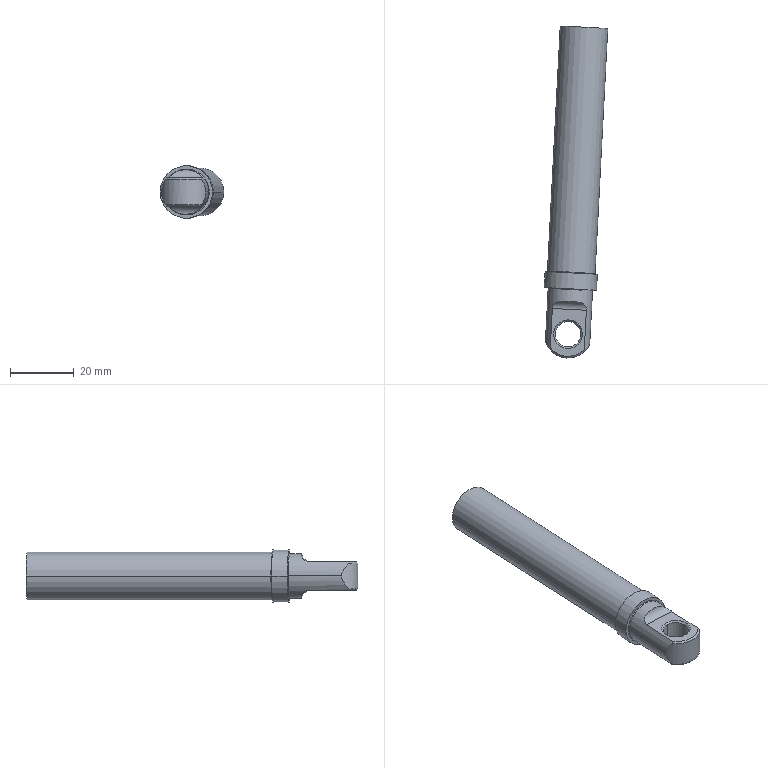Component | SolidWorks | CylinderBarrel-1 | 1 solid | 28 faces | box 20.01 x 104.57 x 16.5 mm | volume 13001 mm3 | cylinder 13 | plane 6 | cone 5 | torus 4 | commonest cylinder face diameters 8 x4 15 x3 14 x2 16.5 x2 5 x2
STEP:
#1=COLOUR_RGB('',0.7922,0.8196,0.9333);
#2=FILL_AREA_STYLE_COLOUR('',#1);
#3=FILL_AREA_STYLE('',(#2));
#4=SURFACE_STYLE_FILL_AREA(#3);
#5=SURFACE_SIDE_STYLE('',(#4));
#6=SURFACE_STYLE_USAGE(.BOTH.,#5);
#7=PRESENTATION_STYLE_ASSIGNMENT((#6));
#8=CARTESIAN_POINT('',(4.187,-5.913,6.691));
#9=VERTEX_POINT('',#8);
#10=CARTESIAN_POINT('',(4.738,-5.942,6.691));
#11=VERTEX_POINT('',#10);
#12=CARTESIAN_POINT('',(4.462,-5.928,6.691));
#13=DIRECTION('',(-0.0519,-0.9987,0.));
#14=DIRECTION('',(0.9987,-0.0519,0.));
#15=AXIS2_PLACEMENT_3D('',#12,#13,#14);
#16=CIRCLE('',#15,0.2756);
#17=EDGE_CURVE('',#9,#11,#16,.T.);
#18=ORIENTED_EDGE('',*,*,#17,.F.);
#19=CARTESIAN_POINT('',(4.178,-5.903,6.691));
#20=VERTEX_POINT('',#19);
#21=CARTESIAN_POINT('',(4.177,-5.913,6.691));
#22=DIRECTION('',(0.,0.,1.));
#23=DIRECTION('',(0.,-1.,0.));
#24=AXIS2_PLACEMENT_3D('',#21,#22,#23);
#25=CIRCLE('',#24,0.009843);
#26=EDGE_CURVE('',#9,#20,#25,.T.);
#27=ORIENTED_EDGE('',*,*,#26,.T.);
#28=CARTESIAN_POINT('',(4.748,-5.933,6.691));
#29=VERTEX_POINT('',#28);
#30=CARTESIAN_POINT('',(4.463,-5.918,6.691));
#31=DIRECTION('',(0.0519,0.9987,-0.));
#32=DIRECTION('',(0.9987,-0.0519,0.));
#33=AXIS2_PLACEMENT_3D('',#30,#31,#32);
#34=CIRCLE('',#33,0.2854);
#35=EDGE_CURVE('',#29,#20,#34,.T.);
#36=ORIENTED_EDGE('',*,*,#35,.F.);
#37=CARTESIAN_POINT('',(4.748,-5.942,6.691));
#38=DIRECTION('',(0.,-0.,-1.));
#39=DIRECTION('',(0.,1.,0.));
#40=AXIS2_PLACEMENT_3D('',#37,#38,#39);
#41=CIRCLE('',#40,0.009843);
#42=EDGE_CURVE('',#11,#29,#41,.T.);
#43=ORIENTED_EDGE('',*,*,#42,.F.);
#44=EDGE_LOOP('',(#18,#27,#36,#43));
#45=FACE_OUTER_BOUND('',#44,.T.);
#46=CARTESIAN_POINT('',(4.462,-5.928,6.691));
#47=DIRECTION('',(-0.0519,-0.9987,0.));
#48=DIRECTION('',(0.9987,-0.0519,-0.));
#49=AXIS2_PLACEMENT_3D('',#46,#47,#48);
#50=TOROIDAL_SURFACE('',#49,0.2854,0.009843);
#51=ADVANCED_FACE('',(#45),#50,.F.);
#52=CARTESIAN_POINT('',(4.168,-5.705,6.691));
#53=VERTEX_POINT('',#52);
#54=CARTESIAN_POINT('',(4.778,-5.737,6.691));
#55=VERTEX_POINT('',#54);
#56=CARTESIAN_POINT('',(4.473,-5.721,6.691));
#57=DIRECTION('',(-0.0519,-0.9987,0.));
#58=DIRECTION('',(0.9987,-0.0519,0.));
#59=AXIS2_PLACEMENT_3D('',#56,#57,#58);
#60=CIRCLE('',#59,0.3051);
#61=EDGE_CURVE('',#53,#55,#60,.T.);
#62=ORIENTED_EDGE('',*,*,#61,.F.);
#63=CARTESIAN_POINT('',(4.179,-5.696,6.691));
#64=VERTEX_POINT('',#63);
#65=CARTESIAN_POINT('',(4.169,-5.696,6.691));
#66=DIRECTION('',(0.,0.,1.));
#67=DIRECTION('',(0.,-1.,0.));
#68=AXIS2_PLACEMENT_3D('',#65,#66,#67);
#69=CIRCLE('',#68,0.009843);
#70=EDGE_CURVE('',#53,#64,#69,.T.);
#71=ORIENTED_EDGE('',*,*,#70,.T.);
#72=CARTESIAN_POINT('',(4.769,-5.727,6.691));
#73=VERTEX_POINT('',#72);
#74=CARTESIAN_POINT('',(4.474,-5.711,6.691));
#75=DIRECTION('',(0.0519,0.9987,-0.));
#76=DIRECTION('',(0.9987,-0.0519,0.));
#77=AXIS2_PLACEMENT_3D('',#74,#75,#76);
#78=CIRCLE('',#77,0.2953);
#79=EDGE_CURVE('',#73,#64,#78,.T.);
#80=ORIENTED_EDGE('',*,*,#79,.F.);
#81=CARTESIAN_POINT('',(4.778,-5.727,6.691));
#82=DIRECTION('',(0.,-0.,-1.));
#83=DIRECTION('',(0.,1.,0.));
#84=AXIS2_PLACEMENT_3D('',#81,#82,#83);
#85=CIRCLE('',#84,0.009843);
#86=EDGE_CURVE('',#55,#73,#85,.T.);
#87=ORIENTED_EDGE('',*,*,#86,.F.);
#88=EDGE_LOOP('',(#62,#71,#80,#87));
#89=FACE_OUTER_BOUND('',#88,.T.);
#90=CARTESIAN_POINT('',(4.474,-5.711,6.691));
#91=DIRECTION('',(-0.0519,-0.9987,0.));
#92=DIRECTION('',(0.9987,-0.0519,0.));
#93=AXIS2_PLACEMENT_3D('',#90,#91,#92);
#94=TOROIDAL_SURFACE('',#93,0.3051,0.009843);
#95=ADVANCED_FACE('',(#89),#94,.F.);
#96=CARTESIAN_POINT('',(4.419,-6.756,6.514));
#97=VERTEX_POINT('',#96);
#98=CARTESIAN_POINT('',(4.214,-6.646,6.514));
#99=VERTEX_POINT('',#98);
#100=CARTESIAN_POINT('',(4.434,-6.48,6.514));
#101=DIRECTION('',(0.,-0.,-1.));
#102=DIRECTION('',(-0.0519,-0.9987,0.));
#103=AXIS2_PLACEMENT_3D('',#100,#101,#102);
#104=CIRCLE('',#103,0.2756);
#105=EDGE_CURVE('',#97,#99,#104,.T.);
#106=ORIENTED_EDGE('',*,*,#105,.F.);
#107=CARTESIAN_POINT('',(4.418,-6.775,6.534));
#108=VERTEX_POINT('',#107);
#109=CARTESIAN_POINT('',(4.419,-6.756,6.514));
#110=DIRECTION('',(-0.0367,-0.7062,0.7071));
#111=VECTOR('',#110,39.37);
#112=LINE('',#109,#111);
#113=EDGE_CURVE('',#97,#108,#112,.T.);
#114=ORIENTED_EDGE('',*,*,#113,.T.);
#115=CARTESIAN_POINT('',(4.198,-6.658,6.534));
#116=VERTEX_POINT('',#115);
#117=CARTESIAN_POINT('',(4.434,-6.48,6.534));
#118=DIRECTION('',(-0.,0.,1.));
#119=DIRECTION('',(-0.0519,-0.9987,0.));
#120=AXIS2_PLACEMENT_3D('',#117,#118,#119);
#121=CIRCLE('',#120,0.2953);
#122=EDGE_CURVE('',#116,#108,#121,.T.);
#123=ORIENTED_EDGE('',*,*,#122,.F.);
#124=CARTESIAN_POINT('',(4.214,-6.646,6.514));
#125=CARTESIAN_POINT('',(4.208,-6.65,6.521));
#126=CARTESIAN_POINT('',(4.203,-6.654,6.527));
#127=CARTESIAN_POINT('',(4.198,-6.658,6.534));
#128=B_SPLINE_CURVE_WITH_KNOTS('',3,(#124,#125,#126,#127),.UNSPECIFIED.,.F.,.F.,(4,4),(0.,0.0007071),.UNSPECIFIED.);
#129=EDGE_CURVE('',#99,#116,#128,.T.);
#130=ORIENTED_EDGE('',*,*,#129,.F.);
#131=EDGE_LOOP('',(#106,#114,#123,#130));
#132=FACE_OUTER_BOUND('',#131,.T.);
#133=CARTESIAN_POINT('',(4.434,-6.48,6.514));
#134=DIRECTION('',(-0.,0.,1.));
#135=DIRECTION('',(-0.0519,-0.9987,0.));
#136=AXIS2_PLACEMENT_3D('',#133,#134,#135);
#137=CONICAL_SURFACE('',#136,0.2756,0.7854);
#138=ADVANCED_FACE('',(#132),#137,.T.);
#139=CARTESIAN_POINT('',(4.442,-6.323,6.849));
#140=VERTEX_POINT('',#139);
#141=CARTESIAN_POINT('',(4.426,-6.638,6.849));
#142=VERTEX_POINT('',#141);
#143=CARTESIAN_POINT('',(4.434,-6.48,6.849));
#144=DIRECTION('',(-0.,0.,1.));
#145=DIRECTION('',(0.0519,0.9987,0.));
#146=AXIS2_PLACEMENT_3D('',#143,#144,#145);
#147=CIRCLE('',#146,0.1575);
#148=EDGE_CURVE('',#140,#142,#147,.T.);
#149=ORIENTED_EDGE('',*,*,#148,.F.);
#150=CARTESIAN_POINT('',(4.443,-6.303,6.869));
#151=VERTEX_POINT('',#150);
#152=CARTESIAN_POINT('',(4.443,-6.303,6.869));
#153=DIRECTION('',(0.0367,0.7062,0.7071));
#154=VECTOR('',#153,39.37);
#155=LINE('',#152,#154);
#156=EDGE_CURVE('',#140,#151,#155,.T.);
#157=ORIENTED_EDGE('',*,*,#156,.T.);
#158=CARTESIAN_POINT('',(4.425,-6.657,6.869));
#159=VERTEX_POINT('',#158);
#160=CARTESIAN_POINT('',(4.434,-6.48,6.869));
#161=DIRECTION('',(0.,-0.,-1.));
#162=DIRECTION('',(0.0519,0.9987,0.));
#163=AXIS2_PLACEMENT_3D('',#160,#161,#162);
#164=CIRCLE('',#163,0.1772);
#165=EDGE_CURVE('',#159,#151,#164,.T.);
#166=ORIENTED_EDGE('',*,*,#165,.F.);
#167=CARTESIAN_POINT('',(4.425,-6.657,6.869));
#168=DIRECTION('',(-0.0367,-0.7062,0.7071));
#169=VECTOR('',#168,39.37);
#170=LINE('',#167,#169);
#171=EDGE_CURVE('',#142,#159,#170,.T.);
#172=ORIENTED_EDGE('',*,*,#171,.F.);
#173=EDGE_LOOP('',(#149,#157,#166,#172));
#174=FACE_OUTER_BOUND('',#173,.T.);
#175=CARTESIAN_POINT('',(4.434,-6.48,6.869));
#176=DIRECTION('',(-0.,0.,1.));
#177=DIRECTION('',(-0.0519,-0.9987,0.));
#178=AXIS2_PLACEMENT_3D('',#175,#176,#177);
#179=CONICAL_SURFACE('',#178,0.1772,0.7854);
#180=ADVANCED_FACE('',(#174),#179,.F.);
#181=CARTESIAN_POINT('',(4.442,-6.323,6.514));
#182=VERTEX_POINT('',#181);
#183=CARTESIAN_POINT('',(4.426,-6.638,6.514));
#184=VERTEX_POINT('',#183);
#185=CARTESIAN_POINT('',(4.434,-6.48,6.514));
#186=DIRECTION('',(-0.,0.,1.));
#187=DIRECTION('',(-0.0519,-0.9987,0.));
#188=AXIS2_PLACEMENT_3D('',#185,#186,#187);
#189=CIRCLE('',#188,0.1575);
#190=EDGE_CURVE('',#182,#184,#189,.T.);
#191=ORIENTED_EDGE('',*,*,#190,.F.);
#192=CARTESIAN_POINT('',(4.442,-6.323,6.298));
#193=DIRECTION('',(-0.,0.,1.));
#194=VECTOR('',#193,39.37);
#195=LINE('',#192,#194);
#196=EDGE_CURVE('',#182,#140,#195,.T.);
#197=ORIENTED_EDGE('',*,*,#196,.T.);
#198=ORIENTED_EDGE('',*,*,#148,.T.);
#199=CARTESIAN_POINT('',(4.426,-6.638,6.298));
#200=DIRECTION('',(-0.,0.,1.));
#201=VECTOR('',#200,39.37);
#202=LINE('',#199,#201);
#203=EDGE_CURVE('',#184,#142,#202,.T.);
#204=ORIENTED_EDGE('',*,*,#203,.F.);
#205=EDGE_LOOP('',(#191,#197,#198,#204));
#206=FACE_OUTER_BOUND('',#205,.T.);
#207=CARTESIAN_POINT('',(4.434,-6.48,6.298));
#208=DIRECTION('',(-0.,0.,1.));
#209=DIRECTION('',(-0.0519,-0.9987,0.));
#210=AXIS2_PLACEMENT_3D('',#207,#208,#209);
#211=CYLINDRICAL_SURFACE('',#210,0.1575);
#212=ADVANCED_FACE('',(#206),#211,.F.);
#213=CARTESIAN_POINT('',(4.65,-6.682,6.849));
#214=VERTEX_POINT('',#213);
#215=CARTESIAN_POINT('',(4.703,-6.6,6.691));
#216=VERTEX_POINT('',#215);
#217=CARTESIAN_POINT('',(4.65,-6.682,6.849));
#218=CARTESIAN_POINT('',(4.658,-6.673,6.838));
#219=CARTESIAN_POINT('',(4.665,-6.665,6.827));
#220=CARTESIAN_POINT('',(4.677,-6.648,6.804));
#221=CARTESIAN_POINT('',(4.683,-6.639,6.792));
#222=CARTESIAN_POINT('',(4.692,-6.623,6.766));
#223=CARTESIAN_POINT('',(4.696,-6.616,6.752));
#224=CARTESIAN_POINT('',(4.7,-6.607,6.73));
#225=CARTESIAN_POINT('',(4.702,-6.605,6.723));
#226=CARTESIAN_POINT('',(4.703,-6.601,6.707));
#227=CARTESIAN_POINT('',(4.703,-6.6,6.699));
#228=CARTESIAN_POINT('',(4.703,-6.6,6.691));
#229=B_SPLINE_CURVE_WITH_KNOTS('',3,(#217,#218,#219,#220,#221,#222,#223,#224,#225,#226,#227,#228),.UNSPECIFIED.,.F.,.F.,(4,2,2,2,2,4),(0.0007506,0.001947,0.003143,0.004339,0.004937,0.005535),.UNSPECIFIED.);
#230=EDGE_CURVE('',#214,#216,#229,.T.);
#231=ORIENTED_EDGE('',*,*,#230,.T.);
#232=CARTESIAN_POINT('',(4.73,-6.089,6.691));
#233=DIRECTION('',(0.0519,0.9987,-0.));
#234=VECTOR('',#233,39.37);
#235=LINE('',#232,#234);
#236=EDGE_CURVE('',#216,#11,#235,.T.);
#237=ORIENTED_EDGE('',*,*,#236,.T.);
#238=CARTESIAN_POINT('',(4.462,-5.928,6.691));
#239=DIRECTION('',(-0.0519,-0.9987,0.));
#240=DIRECTION('',(0.9987,-0.0519,0.));
#241=AXIS2_PLACEMENT_3D('',#238,#239,#240);
#242=CIRCLE('',#241,0.2756);
#243=EDGE_CURVE('',#11,#9,#242,.T.);
#244=ORIENTED_EDGE('',*,*,#243,.T.);
#245=CARTESIAN_POINT('',(4.153,-6.572,6.691));
#246=VERTEX_POINT('',#245);
#247=CARTESIAN_POINT('',(4.18,-6.061,6.691));
#248=DIRECTION('',(0.0519,0.9987,-0.));
#249=VECTOR('',#248,39.37);
#250=LINE('',#247,#249);
#251=EDGE_CURVE('',#246,#9,#250,.T.);
#252=ORIENTED_EDGE('',*,*,#251,.F.);
#253=CARTESIAN_POINT('',(4.198,-6.658,6.849));
#254=VERTEX_POINT('',#253);
#255=CARTESIAN_POINT('',(4.153,-6.572,6.691));
#256=CARTESIAN_POINT('',(4.153,-6.572,6.699));
#257=CARTESIAN_POINT('',(4.153,-6.573,6.707));
#258=CARTESIAN_POINT('',(4.154,-6.576,6.723));
#259=CARTESIAN_POINT('',(4.155,-6.579,6.73));
#260=CARTESIAN_POINT('',(4.159,-6.588,6.752));
#261=CARTESIAN_POINT('',(4.162,-6.595,6.766));
#262=CARTESIAN_POINT('',(4.169,-6.612,6.792));
#263=CARTESIAN_POINT('',(4.174,-6.621,6.804));
#264=CARTESIAN_POINT('',(4.185,-6.64,6.827));
#265=CARTESIAN_POINT('',(4.191,-6.649,6.838));
#266=CARTESIAN_POINT('',(4.198,-6.658,6.849));
#267=B_SPLINE_CURVE_WITH_KNOTS('',3,(#255,#256,#257,#258,#259,#260,#261,#262,#263,#264,#265,#266),.UNSPECIFIED.,.F.,.F.,(4,2,2,2,2,4),(0.005535,0.006132,0.006728,0.007922,0.009116,0.01031),.UNSPECIFIED.);
#268=EDGE_CURVE('',#246,#254,#267,.T.);
#269=ORIENTED_EDGE('',*,*,#268,.T.);
#270=CARTESIAN_POINT('',(4.214,-6.646,6.869));
#271=VERTEX_POINT('',#270);
#272=CARTESIAN_POINT('',(4.198,-6.658,6.849));
#273=CARTESIAN_POINT('',(4.203,-6.654,6.855));
#274=CARTESIAN_POINT('',(4.208,-6.65,6.862));
#275=CARTESIAN_POINT('',(4.214,-6.646,6.869));
#276=B_SPLINE_CURVE_WITH_KNOTS('',3,(#272,#273,#274,#275),.UNSPECIFIED.,.F.,.F.,(4,4),(0.,0.0007071),.UNSPECIFIED.);
#277=EDGE_CURVE('',#254,#271,#276,.T.);
#278=ORIENTED_EDGE('',*,*,#277,.T.);
#279=CARTESIAN_POINT('',(4.239,-6.162,6.869));
#280=VERTEX_POINT('',#279);
#281=CARTESIAN_POINT('',(4.217,-6.575,6.869));
#282=DIRECTION('',(0.0519,0.9987,-0.));
#283=VECTOR('',#282,39.37);
#284=LINE('',#281,#283);
#285=EDGE_CURVE('',#271,#280,#284,.T.);
#286=ORIENTED_EDGE('',*,*,#285,.T.);
#287=CARTESIAN_POINT('',(4.661,-6.184,6.869));
#288=VERTEX_POINT('',#287);
#289=CARTESIAN_POINT('',(4.239,-6.162,6.869));
#290=CARTESIAN_POINT('',(4.239,-6.156,6.869));
#291=CARTESIAN_POINT('',(4.24,-6.15,6.869));
#292=CARTESIAN_POINT('',(4.242,-6.139,6.871));
#293=CARTESIAN_POINT('',(4.244,-6.133,6.873));
#294=CARTESIAN_POINT('',(4.25,-6.117,6.879));
#295=CARTESIAN_POINT('',(4.256,-6.108,6.885));
#296=CARTESIAN_POINT('',(4.267,-6.097,6.895));
#297=CARTESIAN_POINT('',(4.271,-6.094,6.898));
#298=CARTESIAN_POINT('',(4.279,-6.088,6.905));
#299=CARTESIAN_POINT('',(4.284,-6.086,6.908));
#300=CARTESIAN_POINT('',(4.293,-6.082,6.915));
#301=CARTESIAN_POINT('',(4.297,-6.08,6.918));
#302=CARTESIAN_POINT('',(4.307,-6.077,6.925));
#303=CARTESIAN_POINT('',(4.312,-6.076,6.928));
#304=CARTESIAN_POINT('',(4.328,-6.073,6.936));
#305=CARTESIAN_POINT('',(4.339,-6.072,6.942));
#306=CARTESIAN_POINT('',(4.361,-6.071,6.951));
#307=CARTESIAN_POINT('',(4.372,-6.071,6.955));
#308=CARTESIAN_POINT('',(4.395,-6.072,6.961));
#309=CARTESIAN_POINT('',(4.407,-6.073,6.963));
#310=CARTESIAN_POINT('',(4.431,-6.074,6.966));
#311=CARTESIAN_POINT('',(4.443,-6.074,6.967));
#312=CARTESIAN_POINT('',(4.479,-6.076,6.967));
#313=CARTESIAN_POINT('',(4.503,-6.077,6.964));
#314=CARTESIAN_POINT('',(4.537,-6.08,6.955));
#315=CARTESIAN_POINT('',(4.549,-6.081,6.951));
#316=CARTESIAN_POINT('',(4.571,-6.084,6.942));
#317=CARTESIAN_POINT('',(4.581,-6.086,6.936));
#318=CARTESIAN_POINT('',(4.602,-6.092,6.925));
#319=CARTESIAN_POINT('',(4.611,-6.096,6.918));
#320=CARTESIAN_POINT('',(4.628,-6.106,6.905));
#321=CARTESIAN_POINT('',(4.636,-6.112,6.898));
#322=CARTESIAN_POINT('',(4.646,-6.124,6.888));
#323=CARTESIAN_POINT('',(4.648,-6.129,6.885));
#324=CARTESIAN_POINT('',(4.653,-6.139,6.879));
#325=CARTESIAN_POINT('',(4.655,-6.144,6.877));
#326=CARTESIAN_POINT('',(4.658,-6.155,6.873));
#327=CARTESIAN_POINT('',(4.659,-6.16,6.871));
#328=CARTESIAN_POINT('',(4.661,-6.172,6.869));
#329=CARTESIAN_POINT('',(4.661,-6.178,6.869));
#330=CARTESIAN_POINT('',(4.661,-6.184,6.869));
#331=B_SPLINE_CURVE_WITH_KNOTS('',3,(#289,#290,#291,#292,#293,#294,#295,#296,#297,#298,#299,#300,#301,#302,#303,#304,#305,#306,#307,#308,#309,#310,#311,#312,#313,#314,#315,#316,#317,#318,#319,#320,#321,#322,#323,#324,#325,#326,#327,#328,#329,#330),.UNSPECIFIED.,.F.,.F.,(4,2,2,2,2,2,2,2,2,2,2,2,2,2,2,2,2,2,2,2,4),(0.,0.0004585,0.000917,0.001834,0.002292,0.002751,0.003209,0.003668,0.004585,0.005502,0.006419,0.007336,0.00917,0.01009,0.011,0.01192,0.01284,0.0133,0.01375,0.01421,0.01467),.UNSPECIFIED.);
#332=EDGE_CURVE('',#280,#288,#331,.T.);
#333=ORIENTED_EDGE('',*,*,#332,.T.);
#334=CARTESIAN_POINT('',(4.635,-6.668,6.869));
#335=VERTEX_POINT('',#334);
#336=CARTESIAN_POINT('',(4.639,-6.597,6.869));
#337=DIRECTION('',(0.0519,0.9987,-0.));
#338=VECTOR('',#337,39.37);
#339=LINE('',#336,#338);
#340=EDGE_CURVE('',#335,#288,#339,.T.);
#341=ORIENTED_EDGE('',*,*,#340,.F.);
#342=CARTESIAN_POINT('',(4.635,-6.668,6.869));
#343=CARTESIAN_POINT('',(4.641,-6.672,6.862));
#344=CARTESIAN_POINT('',(4.645,-6.677,6.855));
#345=CARTESIAN_POINT('',(4.65,-6.682,6.849));
#346=B_SPLINE_CURVE_WITH_KNOTS('',3,(#342,#343,#344,#345),.UNSPECIFIED.,.F.,.F.,(4,4),(0.,0.0007071),.UNSPECIFIED.);
#347=EDGE_CURVE('',#335,#214,#346,.T.);
#348=ORIENTED_EDGE('',*,*,#347,.T.);
#349=EDGE_LOOP('',(#231,#237,#244,#252,#269,#278,#286,#333,#341,#348));
#350=FACE_OUTER_BOUND('',#349,.T.);
#351=CARTESIAN_POINT('',(4.455,-6.075,6.691));
#352=DIRECTION('',(0.0519,0.9987,-0.));
#353=DIRECTION('',(-0.9987,0.0519,0.));
#354=AXIS2_PLACEMENT_3D('',#351,#352,#353);
#355=CYLINDRICAL_SURFACE('',#354,0.2756);
#356=ADVANCED_FACE('',(#350),#355,.T.);
#357=CARTESIAN_POINT('',(4.787,-5.935,6.691));
#358=VERTEX_POINT('',#357);
#359=CARTESIAN_POINT('',(4.139,-5.901,6.691));
#360=VERTEX_POINT('',#359);
#361=CARTESIAN_POINT('',(4.463,-5.918,6.691));
#362=DIRECTION('',(-0.0519,-0.9987,0.));
#363=DIRECTION('',(0.9987,-0.0519,0.));
#364=AXIS2_PLACEMENT_3D('',#361,#362,#363);
#365=CIRCLE('',#364,0.3248);
#366=EDGE_CURVE('',#358,#360,#365,.T.);
#367=ORIENTED_EDGE('',*,*,#366,.F.);
#368=CARTESIAN_POINT('',(4.798,-5.738,6.691));
#369=VERTEX_POINT('',#368);
#370=CARTESIAN_POINT('',(4.787,-5.935,6.691));
#371=DIRECTION('',(0.0519,0.9987,-0.));
#372=VECTOR('',#371,39.37);
#373=LINE('',#370,#372);
#374=EDGE_CURVE('',#358,#369,#373,.T.);
#375=ORIENTED_EDGE('',*,*,#374,.T.);
#376=CARTESIAN_POINT('',(4.149,-5.704,6.691));
#377=VERTEX_POINT('',#376);
#378=CARTESIAN_POINT('',(4.473,-5.721,6.691));
#379=DIRECTION('',(-0.0519,-0.9987,0.));
#380=DIRECTION('',(0.9987,-0.0519,0.));
#381=AXIS2_PLACEMENT_3D('',#378,#379,#380);
#382=CIRCLE('',#381,0.3248);
#383=EDGE_CURVE('',#369,#377,#382,.T.);
#384=ORIENTED_EDGE('',*,*,#383,.T.);
#385=CARTESIAN_POINT('',(4.139,-5.901,6.691));
#386=DIRECTION('',(0.0519,0.9987,-0.));
#387=VECTOR('',#386,39.37);
#388=LINE('',#385,#387);
#389=EDGE_CURVE('',#360,#377,#388,.T.);
#390=ORIENTED_EDGE('',*,*,#389,.F.);
#391=EDGE_LOOP('',(#367,#375,#384,#390));
#392=FACE_OUTER_BOUND('',#391,.T.);
#393=CARTESIAN_POINT('',(4.463,-5.918,6.691));
#394=DIRECTION('',(0.0519,0.9987,-0.));
#395=DIRECTION('',(-0.9987,0.0519,0.));
#396=AXIS2_PLACEMENT_3D('',#393,#394,#395);
#397=CYLINDRICAL_SURFACE('',#396,0.3248);
#398=ADVANCED_FACE('',(#392),#397,.T.);
#399=CARTESIAN_POINT('',(4.316,-5.713,6.691));
#400=VERTEX_POINT('',#399);
#401=CARTESIAN_POINT('',(4.63,-5.729,6.691));
#402=VERTEX_POINT('',#401);
#403=CARTESIAN_POINT('',(4.473,-5.721,6.691));
#404=DIRECTION('',(-0.0519,-0.9987,0.));
#405=DIRECTION('',(0.9987,-0.0519,0.));
#406=AXIS2_PLACEMENT_3D('',#403,#404,#405);
#407=CIRCLE('',#406,0.1575);
#408=EDGE_CURVE('',#400,#402,#407,.T.);
#409=ORIENTED_EDGE('',*,*,#408,.T.);
#410=CARTESIAN_POINT('',(4.789,-2.682,6.691));
#411=VERTEX_POINT('',#410);
#412=CARTESIAN_POINT('',(4.63,-5.729,6.691));
#413=DIRECTION('',(0.0519,0.9987,-0.));
#414=VECTOR('',#413,39.37);
#415=LINE('',#412,#414);
#416=EDGE_CURVE('',#402,#411,#415,.T.);
#417=ORIENTED_EDGE('',*,*,#416,.T.);
#418=CARTESIAN_POINT('',(4.474,-2.666,6.691));
#419=VERTEX_POINT('',#418);
#420=CARTESIAN_POINT('',(4.632,-2.674,6.691));
#421=DIRECTION('',(-0.0519,-0.9987,0.));
#422=DIRECTION('',(0.9987,-0.0519,0.));
#423=AXIS2_PLACEMENT_3D('',#420,#421,#422);
#424=CIRCLE('',#423,0.1575);
#425=EDGE_CURVE('',#419,#411,#424,.T.);
#426=ORIENTED_EDGE('',*,*,#425,.F.);
#427=CARTESIAN_POINT('',(4.316,-5.713,6.691));
#428=DIRECTION('',(0.0519,0.9987,-0.));
#429=VECTOR('',#428,39.37);
#430=LINE('',#427,#429);
#431=EDGE_CURVE('',#400,#419,#430,.T.);
#432=ORIENTED_EDGE('',*,*,#431,.F.);
#433=EDGE_LOOP('',(#409,#417,#426,#432));
#434=FACE_OUTER_BOUND('',#433,.T.);
#435=CARTESIAN_POINT('',(4.473,-5.721,6.691));
#436=DIRECTION('',(0.0519,0.9987,-0.));
#437=DIRECTION('',(-0.9987,0.0519,0.));
#438=AXIS2_PLACEMENT_3D('',#435,#436,#437);
#439=CYLINDRICAL_SURFACE('',#438,0.1575);
#440=ADVANCED_FACE('',(#434),#439,.F.);
#441=CARTESIAN_POINT('',(4.474,-5.711,6.691));
#442=DIRECTION('',(0.0519,0.9987,-0.));
#443=DIRECTION('',(0.9987,-0.0519,0.));
#444=AXIS2_PLACEMENT_3D('',#441,#442,#443);
#445=CIRCLE('',#444,0.2953);
#446=EDGE_CURVE('',#64,#73,#445,.T.);
#447=ORIENTED_EDGE('',*,*,#446,.T.);
#448=CARTESIAN_POINT('',(4.926,-2.689,6.691));
#449=VERTEX_POINT('',#448);
#450=CARTESIAN_POINT('',(4.768,-5.737,6.691));
#451=DIRECTION('',(0.0519,0.9987,-0.));
#452=VECTOR('',#451,39.37);
#453=LINE('',#450,#452);
#454=EDGE_CURVE('',#73,#449,#453,.T.);
#455=ORIENTED_EDGE('',*,*,#454,.T.);
#456=CARTESIAN_POINT('',(4.337,-2.659,6.691));
#457=VERTEX_POINT('',#456);
#458=CARTESIAN_POINT('',(4.632,-2.674,6.691));
#459=DIRECTION('',(-0.0519,-0.9987,0.));
#460=DIRECTION('',(0.9987,-0.0519,0.));
#461=AXIS2_PLACEMENT_3D('',#458,#459,#460);
#462=CIRCLE('',#461,0.2953);
#463=EDGE_CURVE('',#449,#457,#462,.T.);
#464=ORIENTED_EDGE('',*,*,#463,.T.);
#465=CARTESIAN_POINT('',(4.178,-5.706,6.691));
#466=DIRECTION('',(0.0519,0.9987,-0.));
#467=VECTOR('',#466,39.37);
#468=LINE('',#465,#467);
#469=EDGE_CURVE('',#64,#457,#468,.T.);
#470=ORIENTED_EDGE('',*,*,#469,.F.);
#471=EDGE_LOOP('',(#447,#455,#464,#470));
#472=FACE_OUTER_BOUND('',#471,.T.);
#473=CARTESIAN_POINT('',(4.473,-5.721,6.691));
#474=DIRECTION('',(0.0519,0.9987,-0.));
#475=DIRECTION('',(-0.9987,0.0519,0.));
#476=AXIS2_PLACEMENT_3D('',#473,#474,#475);
#477=CYLINDRICAL_SURFACE('',#476,0.2953);
#478=ADVANCED_FACE('',(#472),#477,.T.);
#479=ORIENTED_EDGE('',*,*,#35,.T.);
#480=CARTESIAN_POINT('',(4.463,-5.918,6.691));
#481=DIRECTION('',(0.0519,0.9987,-0.));
#482=DIRECTION('',(0.9987,-0.0519,0.));
#483=AXIS2_PLACEMENT_3D('',#480,#481,#482);
#484=CIRCLE('',#483,0.2854);
#485=EDGE_CURVE('',#20,#29,#484,.T.);
#486=ORIENTED_EDGE('',*,*,#485,.T.);
#487=EDGE_LOOP('',(#479,#486));
#488=FACE_BOUND('',#487,.T.);
#489=CARTESIAN_POINT('',(4.463,-5.918,6.691));
#490=DIRECTION('',(-0.0519,-0.9987,0.));
#491=DIRECTION('',(0.9987,-0.0519,0.));
#492=AXIS2_PLACEMENT_3D('',#489,#490,#491);
#493=CIRCLE('',#492,0.3248);
#494=EDGE_CURVE('',#360,#358,#493,.T.);
#495=ORIENTED_EDGE('',*,*,#494,.T.);
#496=ORIENTED_EDGE('',*,*,#366,.T.);
#497=EDGE_LOOP('',(#495,#496));
#498=FACE_OUTER_BOUND('',#497,.T.);
#499=CARTESIAN_POINT('',(4.463,-5.918,6.691));
#500=DIRECTION('',(-0.0519,-0.9987,0.));
#501=DIRECTION('',(0.9987,-0.0519,0.));
#502=AXIS2_PLACEMENT_3D('',#499,#500,#501);
#503=PLANE('',#502);
#504=ADVANCED_FACE('',(#488,#498),#503,.T.);
#505=CARTESIAN_POINT('',(4.632,-2.674,6.691));
#506=DIRECTION('',(-0.0519,-0.9987,0.));
#507=DIRECTION('',(0.9987,-0.0519,0.));
#508=AXIS2_PLACEMENT_3D('',#505,#506,#507);
#509=CIRCLE('',#508,0.2953);
#510=EDGE_CURVE('',#457,#449,#509,.T.);
#511=ORIENTED_EDGE('',*,*,#510,.F.);
#512=ORIENTED_EDGE('',*,*,#463,.F.);
#513=EDGE_LOOP('',(#511,#512));
#514=FACE_OUTER_BOUND('',#513,.T.);
#515=ORIENTED_EDGE('',*,*,#425,.T.);
#516=CARTESIAN_POINT('',(4.632,-2.674,6.691));
#517=DIRECTION('',(-0.0519,-0.9987,0.));
#518=DIRECTION('',(0.9987,-0.0519,0.));
#519=AXIS2_PLACEMENT_3D('',#516,#517,#518);
#520=CIRCLE('',#519,0.1575);
#521=EDGE_CURVE('',#411,#419,#520,.T.);
#522=ORIENTED_EDGE('',*,*,#521,.T.);
#523=EDGE_LOOP('',(#515,#522));
#524=FACE_BOUND('',#523,.T.);
#525=CARTESIAN_POINT('',(4.632,-2.674,6.691));
#526=DIRECTION('',(-0.0519,-0.9987,0.));
#527=DIRECTION('',(0.9987,-0.0519,0.));
#528=AXIS2_PLACEMENT_3D('',#525,#526,#527);
#529=PLANE('',#528);
#530=ADVANCED_FACE('',(#514,#524),#529,.F.);
#531=ORIENTED_EDGE('',*,*,#454,.F.);
#532=ORIENTED_EDGE('',*,*,#79,.T.);
#533=ORIENTED_EDGE('',*,*,#469,.T.);
#534=ORIENTED_EDGE('',*,*,#510,.T.);
#535=EDGE_LOOP('',(#531,#532,#533,#534));
#536=FACE_OUTER_BOUND('',#535,.T.);
#537=CARTESIAN_POINT('',(4.473,-5.721,6.691));
#538=DIRECTION('',(0.0519,0.9987,-0.));
#539=DIRECTION('',(-0.9987,0.0519,0.));
#540=AXIS2_PLACEMENT_3D('',#537,#538,#539);
#541=CYLINDRICAL_SURFACE('',#540,0.2953);
#542=ADVANCED_FACE('',(#536),#541,.T.);
#543=ORIENTED_EDGE('',*,*,#416,.F.);
#544=CARTESIAN_POINT('',(4.473,-5.721,6.691));
#545=DIRECTION('',(-0.0519,-0.9987,0.));
#546=DIRECTION('',(0.9987,-0.0519,0.));
#547=AXIS2_PLACEMENT_3D('',#544,#545,#546);
#548=CIRCLE('',#547,0.1575);
#549=EDGE_CURVE('',#402,#400,#548,.T.);
#550=ORIENTED_EDGE('',*,*,#549,.T.);
#551=ORIENTED_EDGE('',*,*,#431,.T.);
#552=ORIENTED_EDGE('',*,*,#521,.F.);
#553=EDGE_LOOP('',(#543,#550,#551,#552));
#554=FACE_OUTER_BOUND('',#553,.T.);
#555=CARTESIAN_POINT('',(4.473,-5.721,6.691));
#556=DIRECTION('',(0.0519,0.9987,-0.));
#557=DIRECTION('',(-0.9987,0.0519,0.));
#558=AXIS2_PLACEMENT_3D('',#555,#556,#557);
#559=CYLINDRICAL_SURFACE('',#558,0.1575);
#560=ADVANCED_FACE('',(#554),#559,.F.);
#561=ORIENTED_EDGE('',*,*,#408,.F.);
#562=ORIENTED_EDGE('',*,*,#549,.F.);
#563=EDGE_LOOP('',(#561,#562));
#564=FACE_OUTER_BOUND('',#563,.T.);
#565=CARTESIAN_POINT('',(4.473,-5.721,6.691));
#566=DIRECTION('',(-0.0519,-0.9987,0.));
#567=DIRECTION('',(0.9987,-0.0519,0.));
#568=AXIS2_PLACEMENT_3D('',#565,#566,#567);
#569=PLANE('',#568);
#570=ADVANCED_FACE('',(#564),#569,.F.);
#571=CARTESIAN_POINT('',(4.473,-5.721,6.691));
#572=DIRECTION('',(-0.0519,-0.9987,0.));
#573=DIRECTION('',(0.9987,-0.0519,0.));
#574=AXIS2_PLACEMENT_3D('',#571,#572,#573);
#575=CIRCLE('',#574,0.3051);
#576=EDGE_CURVE('',#55,#53,#575,.T.);
#577=ORIENTED_EDGE('',*,*,#576,.T.);
#578=ORIENTED_EDGE('',*,*,#61,.T.);
#579=EDGE_LOOP('',(#577,#578));
#580=FACE_BOUND('',#579,.T.);
#581=CARTESIAN_POINT('',(4.473,-5.721,6.691));
#582=DIRECTION('',(-0.0519,-0.9987,0.));
#583=DIRECTION('',(0.9987,-0.0519,0.));
#584=AXIS2_PLACEMENT_3D('',#581,#582,#583);
#585=CIRCLE('',#584,0.3248);
#586=EDGE_CURVE('',#377,#369,#585,.T.);
#587=ORIENTED_EDGE('',*,*,#586,.F.);
#588=ORIENTED_EDGE('',*,*,#383,.F.);
#589=EDGE_LOOP('',(#587,#588));
#590=FACE_OUTER_BOUND('',#589,.T.);
#591=CARTESIAN_POINT('',(4.473,-5.721,6.691));
#592=DIRECTION('',(-0.0519,-0.9987,0.));
#593=DIRECTION('',(0.9987,-0.0519,0.));
#594=AXIS2_PLACEMENT_3D('',#591,#592,#593);
#595=PLANE('',#594);
#596=ADVANCED_FACE('',(#580,#590),#595,.F.);
#597=ORIENTED_EDGE('',*,*,#374,.F.);
#598=ORIENTED_EDGE('',*,*,#494,.F.);
#599=ORIENTED_EDGE('',*,*,#389,.T.);
#600=ORIENTED_EDGE('',*,*,#586,.T.);
#601=EDGE_LOOP('',(#597,#598,#599,#600));
#602=FACE_OUTER_BOUND('',#601,.T.);
#603=CARTESIAN_POINT('',(4.463,-5.918,6.691));
#604=DIRECTION('',(0.0519,0.9987,-0.));
#605=DIRECTION('',(-0.9987,0.0519,0.));
#606=AXIS2_PLACEMENT_3D('',#603,#604,#605);
#607=CYLINDRICAL_SURFACE('',#606,0.3248);
#608=ADVANCED_FACE('',(#602),#607,.T.);
#609=ORIENTED_EDGE('',*,*,#236,.F.);
#610=CARTESIAN_POINT('',(4.65,-6.682,6.534));
#611=VERTEX_POINT('',#610);
#612=CARTESIAN_POINT('',(4.703,-6.6,6.691));
#613=CARTESIAN_POINT('',(4.703,-6.6,6.683));
#614=CARTESIAN_POINT('',(4.703,-6.601,6.675));
#615=CARTESIAN_POINT('',(4.702,-6.605,6.66));
#616=CARTESIAN_POINT('',(4.7,-6.607,6.652));
#617=CARTESIAN_POINT('',(4.696,-6.616,6.631));
#618=CARTESIAN_POINT('',(4.692,-6.623,6.617));
#619=CARTESIAN_POINT('',(4.683,-6.639,6.591));
#620=CARTESIAN_POINT('',(4.677,-6.647,6.579));
#621=CARTESIAN_POINT('',(4.665,-6.665,6.556));
#622=CARTESIAN_POINT('',(4.658,-6.673,6.545));
#623=CARTESIAN_POINT('',(4.65,-6.682,6.534));
#624=B_SPLINE_CURVE_WITH_KNOTS('',3,(#612,#613,#614,#615,#616,#617,#618,#619,#620,#621,#622,#623),.UNSPECIFIED.,.F.,.F.,(4,2,2,2,2,4),(0.005535,0.006132,0.006728,0.007922,0.009116,0.01031),.UNSPECIFIED.);
#625=EDGE_CURVE('',#216,#611,#624,.T.);
#626=ORIENTED_EDGE('',*,*,#625,.T.);
#627=CARTESIAN_POINT('',(4.635,-6.668,6.514));
#628=VERTEX_POINT('',#627);
#629=CARTESIAN_POINT('',(4.65,-6.682,6.534));
#630=CARTESIAN_POINT('',(4.645,-6.677,6.527));
#631=CARTESIAN_POINT('',(4.641,-6.672,6.521));
#632=CARTESIAN_POINT('',(4.635,-6.668,6.514));
#633=B_SPLINE_CURVE_WITH_KNOTS('',3,(#629,#630,#631,#632),.UNSPECIFIED.,.F.,.F.,(4,4),(0.,0.0007071),.UNSPECIFIED.);
#634=EDGE_CURVE('',#611,#628,#633,.T.);
#635=ORIENTED_EDGE('',*,*,#634,.T.);
#636=CARTESIAN_POINT('',(4.661,-6.184,6.514));
#637=VERTEX_POINT('',#636);
#638=CARTESIAN_POINT('',(4.639,-6.597,6.514));
#639=DIRECTION('',(0.0519,0.9987,-0.));
#640=VECTOR('',#639,39.37);
#641=LINE('',#638,#640);
#642=EDGE_CURVE('',#628,#637,#641,.T.);
#643=ORIENTED_EDGE('',*,*,#642,.T.);
#644=CARTESIAN_POINT('',(4.239,-6.162,6.514));
#645=VERTEX_POINT('',#644);
#646=CARTESIAN_POINT('',(4.661,-6.184,6.514));
#647=CARTESIAN_POINT('',(4.661,-6.178,6.514));
#648=CARTESIAN_POINT('',(4.661,-6.172,6.514));
#649=CARTESIAN_POINT('',(4.659,-6.16,6.512));
#650=CARTESIAN_POINT('',(4.658,-6.155,6.51));
#651=CARTESIAN_POINT('',(4.654,-6.138,6.504));
#652=CARTESIAN_POINT('',(4.649,-6.128,6.498));
#653=CARTESIAN_POINT('',(4.639,-6.116,6.488));
#654=CARTESIAN_POINT('',(4.636,-6.113,6.485));
#655=CARTESIAN_POINT('',(4.628,-6.106,6.478));
#656=CARTESIAN_POINT('',(4.624,-6.103,6.475));
#657=CARTESIAN_POINT('',(4.615,-6.098,6.468));
#658=CARTESIAN_POINT('',(4.611,-6.096,6.465));
#659=CARTESIAN_POINT('',(4.601,-6.092,6.458));
#660=CARTESIAN_POINT('',(4.596,-6.091,6.455));
#661=CARTESIAN_POINT('',(4.581,-6.086,6.447));
#662=CARTESIAN_POINT('',(4.571,-6.084,6.441));
#663=CARTESIAN_POINT('',(4.549,-6.081,6.432));
#664=CARTESIAN_POINT('',(4.537,-6.08,6.428));
#665=CARTESIAN_POINT('',(4.514,-6.078,6.422));
#666=CARTESIAN_POINT('',(4.503,-6.078,6.42));
#667=CARTESIAN_POINT('',(4.479,-6.076,6.417));
#668=CARTESIAN_POINT('',(4.467,-6.076,6.416));
#669=CARTESIAN_POINT('',(4.43,-6.074,6.416));
#670=CARTESIAN_POINT('',(4.407,-6.072,6.419));
#671=CARTESIAN_POINT('',(4.372,-6.071,6.428));
#672=CARTESIAN_POINT('',(4.361,-6.071,6.432));
#673=CARTESIAN_POINT('',(4.338,-6.072,6.441));
#674=CARTESIAN_POINT('',(4.328,-6.073,6.447));
#675=CARTESIAN_POINT('',(4.307,-6.077,6.458));
#676=CARTESIAN_POINT('',(4.297,-6.08,6.465));
#677=CARTESIAN_POINT('',(4.279,-6.088,6.478));
#678=CARTESIAN_POINT('',(4.271,-6.093,6.485));
#679=CARTESIAN_POINT('',(4.26,-6.104,6.495));
#680=CARTESIAN_POINT('',(4.257,-6.109,6.498));
#681=CARTESIAN_POINT('',(4.251,-6.118,6.503));
#682=CARTESIAN_POINT('',(4.248,-6.123,6.506));
#683=CARTESIAN_POINT('',(4.244,-6.133,6.51));
#684=CARTESIAN_POINT('',(4.242,-6.139,6.512));
#685=CARTESIAN_POINT('',(4.24,-6.15,6.514));
#686=CARTESIAN_POINT('',(4.239,-6.156,6.514));
#687=CARTESIAN_POINT('',(4.239,-6.162,6.514));
#688=B_SPLINE_CURVE_WITH_KNOTS('',3,(#646,#647,#648,#649,#650,#651,#652,#653,#654,#655,#656,#657,#658,#659,#660,#661,#662,#663,#664,#665,#666,#667,#668,#669,#670,#671,#672,#673,#674,#675,#676,#677,#678,#679,#680,#681,#682,#683,#684,#685,#686,#687),.UNSPECIFIED.,.F.,.F.,(4,2,2,2,2,2,2,2,2,2,2,2,2,2,2,2,2,2,2,2,4),(0.,0.0004585,0.000917,0.001834,0.002292,0.002751,0.003209,0.003668,0.004585,0.005502,0.006419,0.007336,0.00917,0.01009,0.011,0.01192,0.01284,0.0133,0.01375,0.01421,0.01467),.UNSPECIFIED.);
#689=EDGE_CURVE('',#637,#645,#688,.T.);
#690=ORIENTED_EDGE('',*,*,#689,.T.);
#691=CARTESIAN_POINT('',(4.217,-6.575,6.514));
#692=DIRECTION('',(0.0519,0.9987,-0.));
#693=VECTOR('',#692,39.37);
#694=LINE('',#691,#693);
#695=EDGE_CURVE('',#99,#645,#694,.T.);
#696=ORIENTED_EDGE('',*,*,#695,.F.);
#697=ORIENTED_EDGE('',*,*,#129,.T.);
#698=CARTESIAN_POINT('',(4.198,-6.658,6.534));
#699=CARTESIAN_POINT('',(4.191,-6.649,6.545));
#700=CARTESIAN_POINT('',(4.185,-6.64,6.556));
#701=CARTESIAN_POINT('',(4.174,-6.621,6.579));
#702=CARTESIAN_POINT('',(4.17,-6.612,6.591));
#703=CARTESIAN_POINT('',(4.162,-6.596,6.617));
#704=CARTESIAN_POINT('',(4.159,-6.588,6.63));
#705=CARTESIAN_POINT('',(4.155,-6.579,6.652));
#706=CARTESIAN_POINT('',(4.154,-6.576,6.66));
#707=CARTESIAN_POINT('',(4.153,-6.573,6.676));
#708=CARTESIAN_POINT('',(4.153,-6.572,6.683));
#709=CARTESIAN_POINT('',(4.153,-6.572,6.691));
#710=B_SPLINE_CURVE_WITH_KNOTS('',3,(#698,#699,#700,#701,#702,#703,#704,#705,#706,#707,#708,#709),.UNSPECIFIED.,.F.,.F.,(4,2,2,2,2,4),(0.0007506,0.001947,0.003143,0.004339,0.004937,0.005535),.UNSPECIFIED.);
#711=EDGE_CURVE('',#116,#246,#710,.T.);
#712=ORIENTED_EDGE('',*,*,#711,.T.);
#713=ORIENTED_EDGE('',*,*,#251,.T.);
#714=ORIENTED_EDGE('',*,*,#17,.T.);
#715=EDGE_LOOP('',(#609,#626,#635,#643,#690,#696,#697,#712,#713,#714));
#716=FACE_OUTER_BOUND('',#715,.T.);
#717=CARTESIAN_POINT('',(4.455,-6.075,6.691));
#718=DIRECTION('',(0.0519,0.9987,-0.));
#719=DIRECTION('',(-0.9987,0.0519,0.));
#720=AXIS2_PLACEMENT_3D('',#717,#718,#719);
#721=CYLINDRICAL_SURFACE('',#720,0.2756);
#722=ADVANCED_FACE('',(#716),#721,.T.);
#723=CARTESIAN_POINT('',(4.434,-6.48,6.514));
#724=DIRECTION('',(-0.,0.,1.));
#725=DIRECTION('',(-0.0519,-0.9987,0.));
#726=AXIS2_PLACEMENT_3D('',#723,#724,#725);
#727=CIRCLE('',#726,0.1575);
#728=EDGE_CURVE('',#184,#182,#727,.T.);
#729=ORIENTED_EDGE('',*,*,#728,.T.);
#730=ORIENTED_EDGE('',*,*,#190,.T.);
#731=EDGE_LOOP('',(#729,#730));
#732=FACE_BOUND('',#731,.T.);
#733=ORIENTED_EDGE('',*,*,#642,.F.);
#734=CARTESIAN_POINT('',(4.434,-6.48,6.514));
#735=DIRECTION('',(0.,-0.,-1.));
#736=DIRECTION('',(-0.0519,-0.9987,0.));
#737=AXIS2_PLACEMENT_3D('',#734,#735,#736);
#738=CIRCLE('',#737,0.2756);
#739=EDGE_CURVE('',#628,#97,#738,.T.);
#740=ORIENTED_EDGE('',*,*,#739,.T.);
#741=ORIENTED_EDGE('',*,*,#105,.T.);
#742=ORIENTED_EDGE('',*,*,#695,.T.);
#743=CARTESIAN_POINT('',(4.239,-6.162,6.514));
#744=DIRECTION('',(0.9987,-0.0519,0.));
#745=VECTOR('',#744,39.37);
#746=LINE('',#743,#745);
#747=EDGE_CURVE('',#645,#637,#746,.T.);
#748=ORIENTED_EDGE('',*,*,#747,.T.);
#749=EDGE_LOOP('',(#733,#740,#741,#742,#748));
#750=FACE_OUTER_BOUND('',#749,.T.);
#751=CARTESIAN_POINT('',(4.217,-6.575,6.514));
#752=DIRECTION('',(-0.,0.,1.));
#753=DIRECTION('',(-0.0519,-0.9987,0.));
#754=AXIS2_PLACEMENT_3D('',#751,#752,#753);
#755=PLANE('',#754);
#756=ADVANCED_FACE('',(#732,#750),#755,.F.);
#757=ORIENTED_EDGE('',*,*,#165,.T.);
#758=CARTESIAN_POINT('',(4.434,-6.48,6.869));
#759=DIRECTION('',(0.,-0.,-1.));
#760=DIRECTION('',(0.0519,0.9987,0.));
#761=AXIS2_PLACEMENT_3D('',#758,#759,#760);
#762=CIRCLE('',#761,0.1772);
#763=EDGE_CURVE('',#151,#159,#762,.T.);
#764=ORIENTED_EDGE('',*,*,#763,.T.);
#765=EDGE_LOOP('',(#757,#764));
#766=FACE_BOUND('',#765,.T.);
#767=ORIENTED_EDGE('',*,*,#285,.F.);
#768=CARTESIAN_POINT('',(4.434,-6.48,6.869));
#769=DIRECTION('',(-0.,0.,1.));
#770=DIRECTION('',(0.0519,0.9987,0.));
#771=AXIS2_PLACEMENT_3D('',#768,#769,#770);
#772=CIRCLE('',#771,0.2756);
#773=EDGE_CURVE('',#271,#335,#772,.T.);
#774=ORIENTED_EDGE('',*,*,#773,.T.);
#775=ORIENTED_EDGE('',*,*,#340,.T.);
#776=CARTESIAN_POINT('',(4.239,-6.162,6.869));
#777=DIRECTION('',(-0.9987,0.0519,-0.));
#778=VECTOR('',#777,39.37);
#779=LINE('',#776,#778);
#780=EDGE_CURVE('',#288,#280,#779,.T.);
#781=ORIENTED_EDGE('',*,*,#780,.T.);
#782=EDGE_LOOP('',(#767,#774,#775,#781));
#783=FACE_OUTER_BOUND('',#782,.T.);
#784=CARTESIAN_POINT('',(4.217,-6.575,6.869));
#785=DIRECTION('',(0.,-0.,-1.));
#786=DIRECTION('',(0.0519,0.9987,-0.));
#787=AXIS2_PLACEMENT_3D('',#784,#785,#786);
#788=PLANE('',#787);
#789=ADVANCED_FACE('',(#766,#783),#788,.F.);
#790=ORIENTED_EDGE('',*,*,#230,.F.);
#791=CARTESIAN_POINT('',(4.434,-6.48,6.849));
#792=DIRECTION('',(0.,-0.,-1.));
#793=DIRECTION('',(0.0519,0.9987,0.));
#794=AXIS2_PLACEMENT_3D('',#791,#792,#793);
#795=CIRCLE('',#794,0.2953);
#796=EDGE_CURVE('',#214,#254,#795,.T.);
#797=ORIENTED_EDGE('',*,*,#796,.T.);
#798=ORIENTED_EDGE('',*,*,#268,.F.);
#799=ORIENTED_EDGE('',*,*,#711,.F.);
#800=ORIENTED_EDGE('',*,*,#122,.T.);
#801=CARTESIAN_POINT('',(4.434,-6.48,6.534));
#802=DIRECTION('',(-0.,0.,1.));
#803=DIRECTION('',(-0.0519,-0.9987,0.));
#804=AXIS2_PLACEMENT_3D('',#801,#802,#803);
#805=CIRCLE('',#804,0.2953);
#806=EDGE_CURVE('',#108,#611,#805,.T.);
#807=ORIENTED_EDGE('',*,*,#806,.T.);
#808=ORIENTED_EDGE('',*,*,#625,.F.);
#809=EDGE_LOOP('',(#790,#797,#798,#799,#800,#807,#808));
#810=FACE_OUTER_BOUND('',#809,.T.);
#811=CARTESIAN_POINT('',(4.434,-6.48,7.085));
#812=DIRECTION('',(0.,-0.,-1.));
#813=DIRECTION('',(0.0519,0.9987,0.));
#814=AXIS2_PLACEMENT_3D('',#811,#812,#813);
#815=CYLINDRICAL_SURFACE('',#814,0.2953);
#816=ADVANCED_FACE('',(#810),#815,.T.);
#817=ORIENTED_EDGE('',*,*,#196,.F.);
#818=ORIENTED_EDGE('',*,*,#728,.F.);
#819=ORIENTED_EDGE('',*,*,#203,.T.);
#820=CARTESIAN_POINT('',(4.434,-6.48,6.849));
#821=DIRECTION('',(-0.,0.,1.));
#822=DIRECTION('',(0.0519,0.9987,0.));
#823=AXIS2_PLACEMENT_3D('',#820,#821,#822);
#824=CIRCLE('',#823,0.1575);
#825=EDGE_CURVE('',#142,#140,#824,.T.);
#826=ORIENTED_EDGE('',*,*,#825,.T.);
#827=EDGE_LOOP('',(#817,#818,#819,#826));
#828=FACE_OUTER_BOUND('',#827,.T.);
#829=CARTESIAN_POINT('',(4.434,-6.48,6.298));
#830=DIRECTION('',(-0.,0.,1.));
#831=DIRECTION('',(-0.0519,-0.9987,0.));
#832=AXIS2_PLACEMENT_3D('',#829,#830,#831);
#833=CYLINDRICAL_SURFACE('',#832,0.1575);
#834=ADVANCED_FACE('',(#828),#833,.F.);
#835=ORIENTED_EDGE('',*,*,#780,.F.);
#836=ORIENTED_EDGE('',*,*,#332,.F.);
#837=EDGE_LOOP('',(#835,#836));
#838=FACE_OUTER_BOUND('',#837,.T.);
#839=CARTESIAN_POINT('',(4.239,-6.162,6.967));
#840=DIRECTION('',(-0.9987,0.0519,-0.));
#841=DIRECTION('',(-0.0519,-0.9987,0.));
#842=AXIS2_PLACEMENT_3D('',#839,#840,#841);
#843=CYLINDRICAL_SURFACE('',#842,0.09843);
#844=ADVANCED_FACE('',(#838),#843,.F.);
#845=ORIENTED_EDGE('',*,*,#747,.F.);
#846=ORIENTED_EDGE('',*,*,#689,.F.);
#847=EDGE_LOOP('',(#845,#846));
#848=FACE_OUTER_BOUND('',#847,.T.);
#849=CARTESIAN_POINT('',(4.239,-6.162,6.416));
#850=DIRECTION('',(0.9987,-0.0519,0.));
#851=DIRECTION('',(0.0519,0.9987,0.));
#852=AXIS2_PLACEMENT_3D('',#849,#850,#851);
#853=CYLINDRICAL_SURFACE('',#852,0.09843);
#854=ADVANCED_FACE('',(#848),#853,.F.);
#855=ORIENTED_EDGE('',*,*,#156,.F.);
#856=ORIENTED_EDGE('',*,*,#825,.F.);
#857=ORIENTED_EDGE('',*,*,#171,.T.);
#858=ORIENTED_EDGE('',*,*,#763,.F.);
#859=EDGE_LOOP('',(#855,#856,#857,#858));
#860=FACE_OUTER_BOUND('',#859,.T.);
#861=CARTESIAN_POINT('',(4.434,-6.48,6.869));
#862=DIRECTION('',(-0.,0.,1.));
#863=DIRECTION('',(-0.0519,-0.9987,0.));
#864=AXIS2_PLACEMENT_3D('',#861,#862,#863);
#865=CONICAL_SURFACE('',#864,0.1772,0.7854);
#866=ADVANCED_FACE('',(#860),#865,.F.);
#867=ORIENTED_EDGE('',*,*,#277,.F.);
#868=ORIENTED_EDGE('',*,*,#796,.F.);
#869=ORIENTED_EDGE('',*,*,#347,.F.);
#870=ORIENTED_EDGE('',*,*,#773,.F.);
#871=EDGE_LOOP('',(#867,#868,#869,#870));
#872=FACE_OUTER_BOUND('',#871,.T.);
#873=CARTESIAN_POINT('',(4.434,-6.48,6.869));
#874=DIRECTION('',(0.,-0.,-1.));
#875=DIRECTION('',(0.0519,0.9987,0.));
#876=AXIS2_PLACEMENT_3D('',#873,#874,#875);
#877=CONICAL_SURFACE('',#876,0.2756,0.7854);
#878=ADVANCED_FACE('',(#872),#877,.T.);
#879=ORIENTED_EDGE('',*,*,#113,.F.);
#880=ORIENTED_EDGE('',*,*,#739,.F.);
#881=ORIENTED_EDGE('',*,*,#634,.F.);
#882=ORIENTED_EDGE('',*,*,#806,.F.);
#883=EDGE_LOOP('',(#879,#880,#881,#882));
#884=FACE_OUTER_BOUND('',#883,.T.);
#885=CARTESIAN_POINT('',(4.434,-6.48,6.514));
#886=DIRECTION('',(-0.,0.,1.));
#887=DIRECTION('',(-0.0519,-0.9987,0.));
#888=AXIS2_PLACEMENT_3D('',#885,#886,#887);
#889=CONICAL_SURFACE('',#888,0.2756,0.7854);
#890=ADVANCED_FACE('',(#884),#889,.T.);
#891=ORIENTED_EDGE('',*,*,#70,.F.);
#892=ORIENTED_EDGE('',*,*,#576,.F.);
#893=ORIENTED_EDGE('',*,*,#86,.T.);
#894=ORIENTED_EDGE('',*,*,#446,.F.);
#895=EDGE_LOOP('',(#891,#892,#893,#894));
#896=FACE_OUTER_BOUND('',#895,.T.);
#897=CARTESIAN_POINT('',(4.474,-5.711,6.691));
#898=DIRECTION('',(-0.0519,-0.9987,0.));
#899=DIRECTION('',(0.9987,-0.0519,0.));
#900=AXIS2_PLACEMENT_3D('',#897,#898,#899);
#901=TOROIDAL_SURFACE('',#900,0.3051,0.009843);
#902=ADVANCED_FACE('',(#896),#901,.F.);
#903=ORIENTED_EDGE('',*,*,#26,.F.);
#904=ORIENTED_EDGE('',*,*,#243,.F.);
#905=ORIENTED_EDGE('',*,*,#42,.T.);
#906=ORIENTED_EDGE('',*,*,#485,.F.);
#907=EDGE_LOOP('',(#903,#904,#905,#906));
#908=FACE_OUTER_BOUND('',#907,.T.);
#909=CARTESIAN_POINT('',(4.462,-5.928,6.691));
#910=DIRECTION('',(-0.0519,-0.9987,0.));
#911=DIRECTION('',(0.9987,-0.0519,-0.));
#912=AXIS2_PLACEMENT_3D('',#909,#910,#911);
#913=TOROIDAL_SURFACE('',#912,0.2854,0.009843);
#914=ADVANCED_FACE('',(#908),#913,.F.);
#915=CLOSED_SHELL('',(#51,#95,#138,#180,#212,#356,#398,#440,#478,#504,#530,#542,#560,#570,#596,#608,#722,#756,#789,#816,#834,#844,#854,#866,#878,#890,#902,#914));
#916=MANIFOLD_SOLID_BREP('',#915);
#917=STYLED_ITEM('',(#7),#916);
#918=(LENGTH_UNIT()NAMED_UNIT(*)SI_UNIT($,.METRE.));
#919=LENGTH_MEASURE_WITH_UNIT(LENGTH_MEASURE(0.0254),#918);
#920=DIMENSIONAL_EXPONENTS(1.,0.,0.,0.,0.,0.,0.);
#921=(CONVERSION_BASED_UNIT('',#919)LENGTH_UNIT()NAMED_UNIT(#920));
#922=UNCERTAINTY_MEASURE_WITH_UNIT(LENGTH_MEASURE(0.00001),#921,'','');
#923=(NAMED_UNIT(*)PLANE_ANGLE_UNIT()SI_UNIT($,.RADIAN.));
#924=(NAMED_UNIT(*)SI_UNIT($,.STERADIAN.)SOLID_ANGLE_UNIT());
#925=(GEOMETRIC_REPRESENTATION_CONTEXT(3)GLOBAL_UNCERTAINTY_ASSIGNED_CONTEXT((#922))GLOBAL_UNIT_ASSIGNED_CONTEXT((#921,#923,#924))REPRESENTATION_CONTEXT('',''));
#926=MECHANICAL_DESIGN_GEOMETRIC_PRESENTATION_REPRESENTATION('',(#917),#925);
#927=CARTESIAN_POINT('',(0.,0.,0.));
#928=DIRECTION('',(0.,0.,1.));
#929=DIRECTION('',(1.,0.,0.));
#930=AXIS2_PLACEMENT_3D('',#927,#928,#929);
#931=(LENGTH_UNIT()NAMED_UNIT(*)SI_UNIT($,.METRE.));
#932=LENGTH_MEASURE_WITH_UNIT(LENGTH_MEASURE(0.0254),#931);
#933=DIMENSIONAL_EXPONENTS(1.,0.,0.,0.,0.,0.,0.);
#934=(CONVERSION_BASED_UNIT('',#932)LENGTH_UNIT()NAMED_UNIT(#933));
#935=UNCERTAINTY_MEASURE_WITH_UNIT(LENGTH_MEASURE(0.00001),#934,'','');
#936=(NAMED_UNIT(*)PLANE_ANGLE_UNIT()SI_UNIT($,.RADIAN.));
#937=(NAMED_UNIT(*)SI_UNIT($,.STERADIAN.)SOLID_ANGLE_UNIT());
#938=(GEOMETRIC_REPRESENTATION_CONTEXT(3)GLOBAL_UNCERTAINTY_ASSIGNED_CONTEXT((#935))GLOBAL_UNIT_ASSIGNED_CONTEXT((#934,#936,#937))REPRESENTATION_CONTEXT('',''));
#939=ADVANCED_BREP_SHAPE_REPRESENTATION('',(#916,#930),#938);
#940=PRESENTATION_LAYER_ASSIGNMENT('','',(#917));